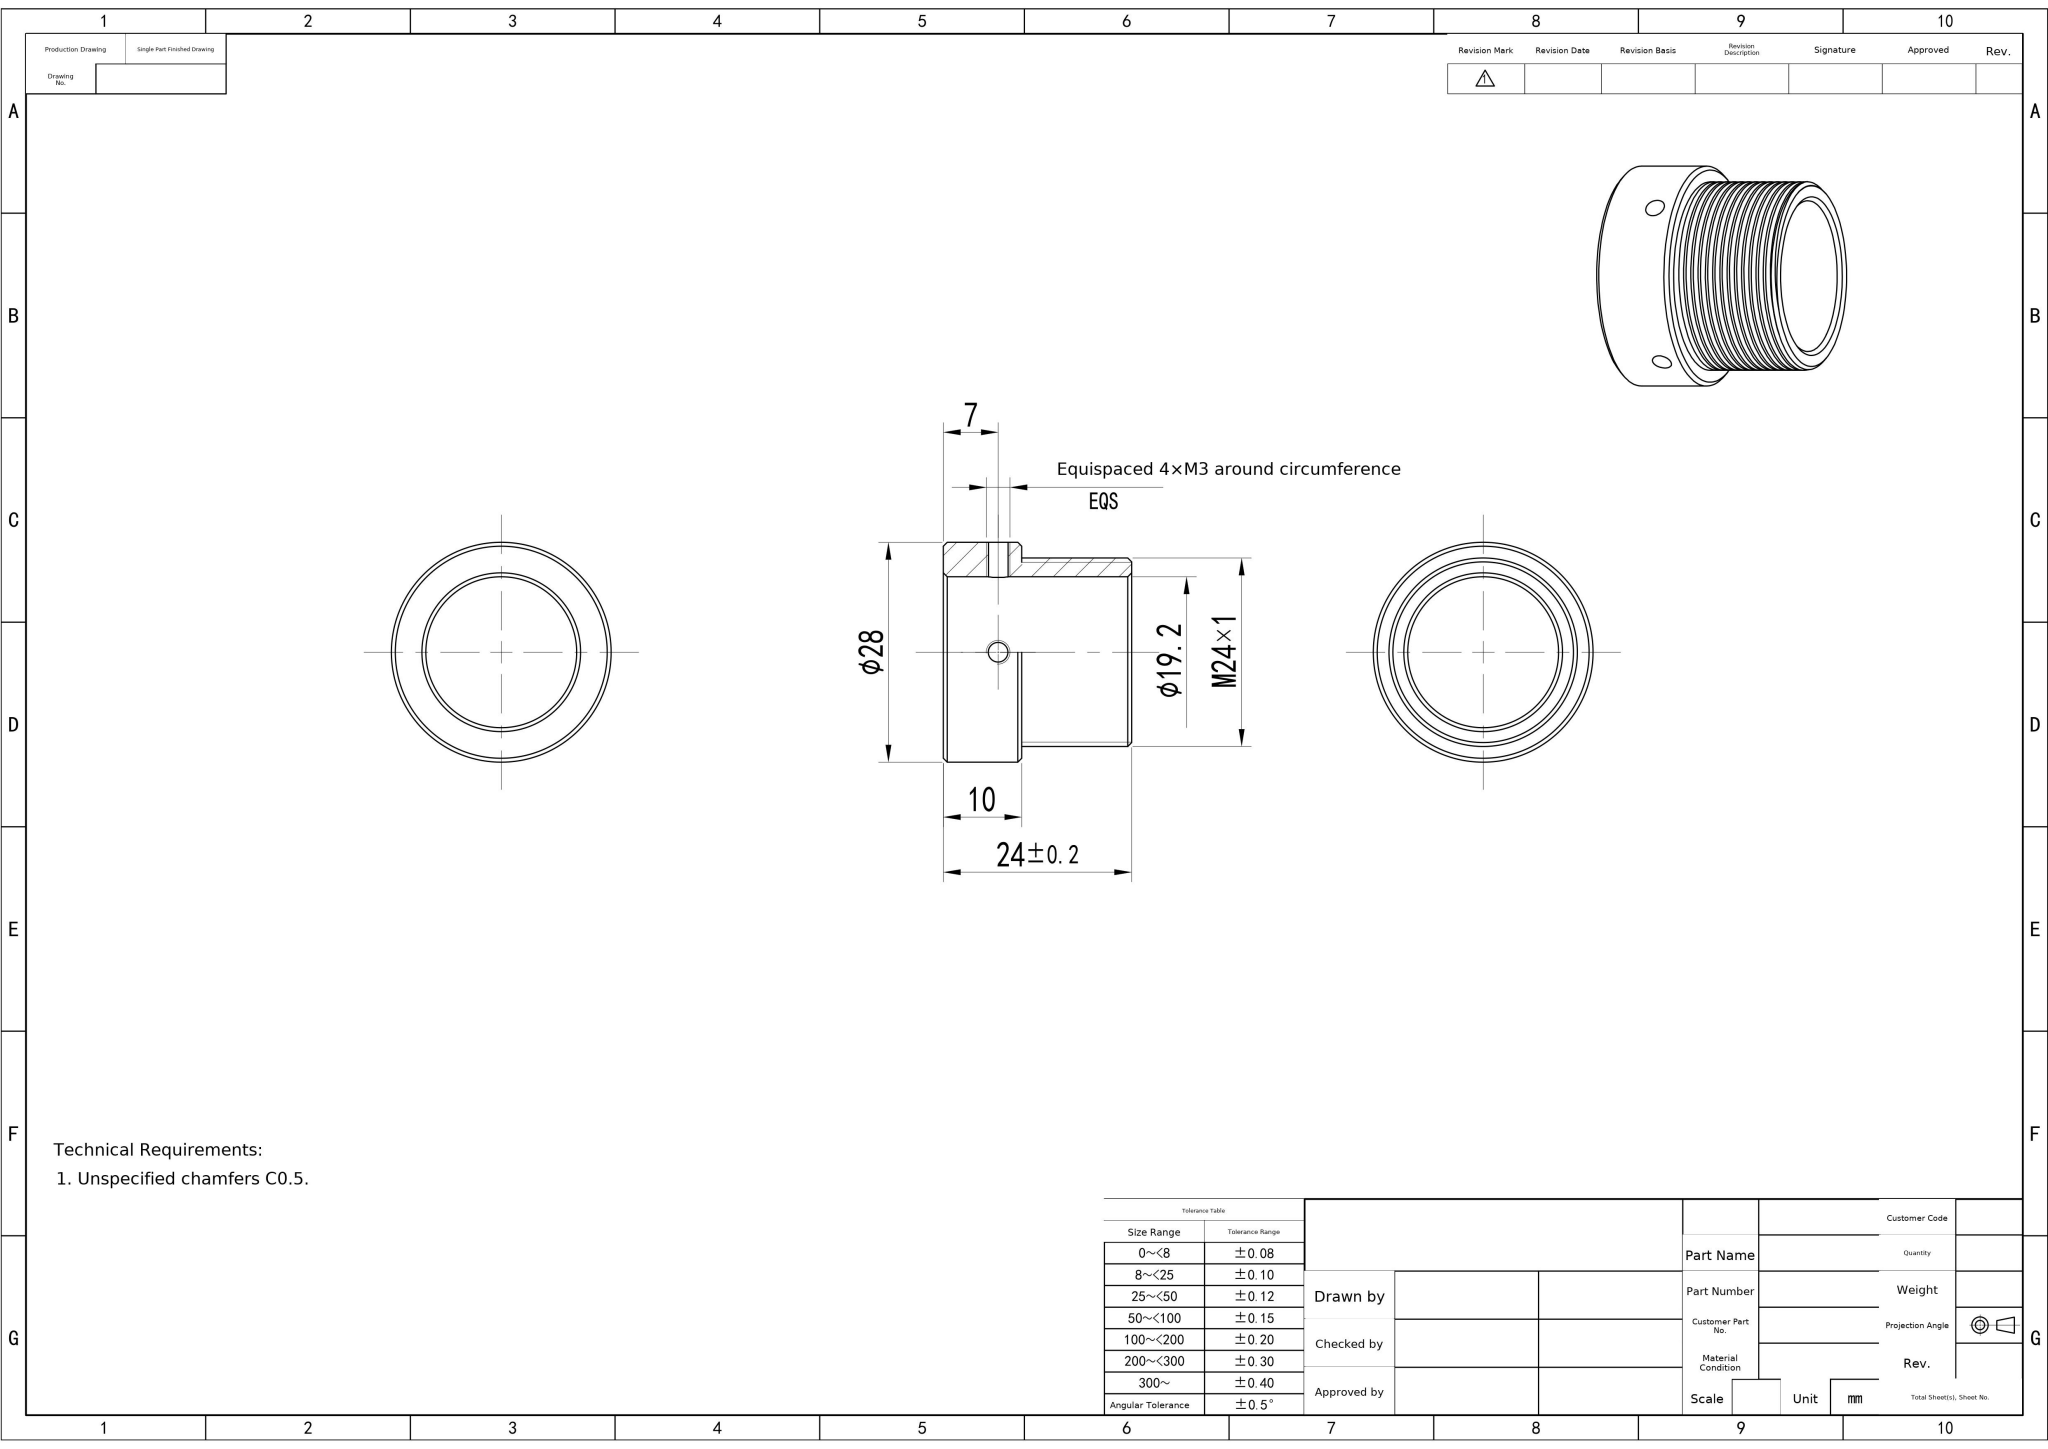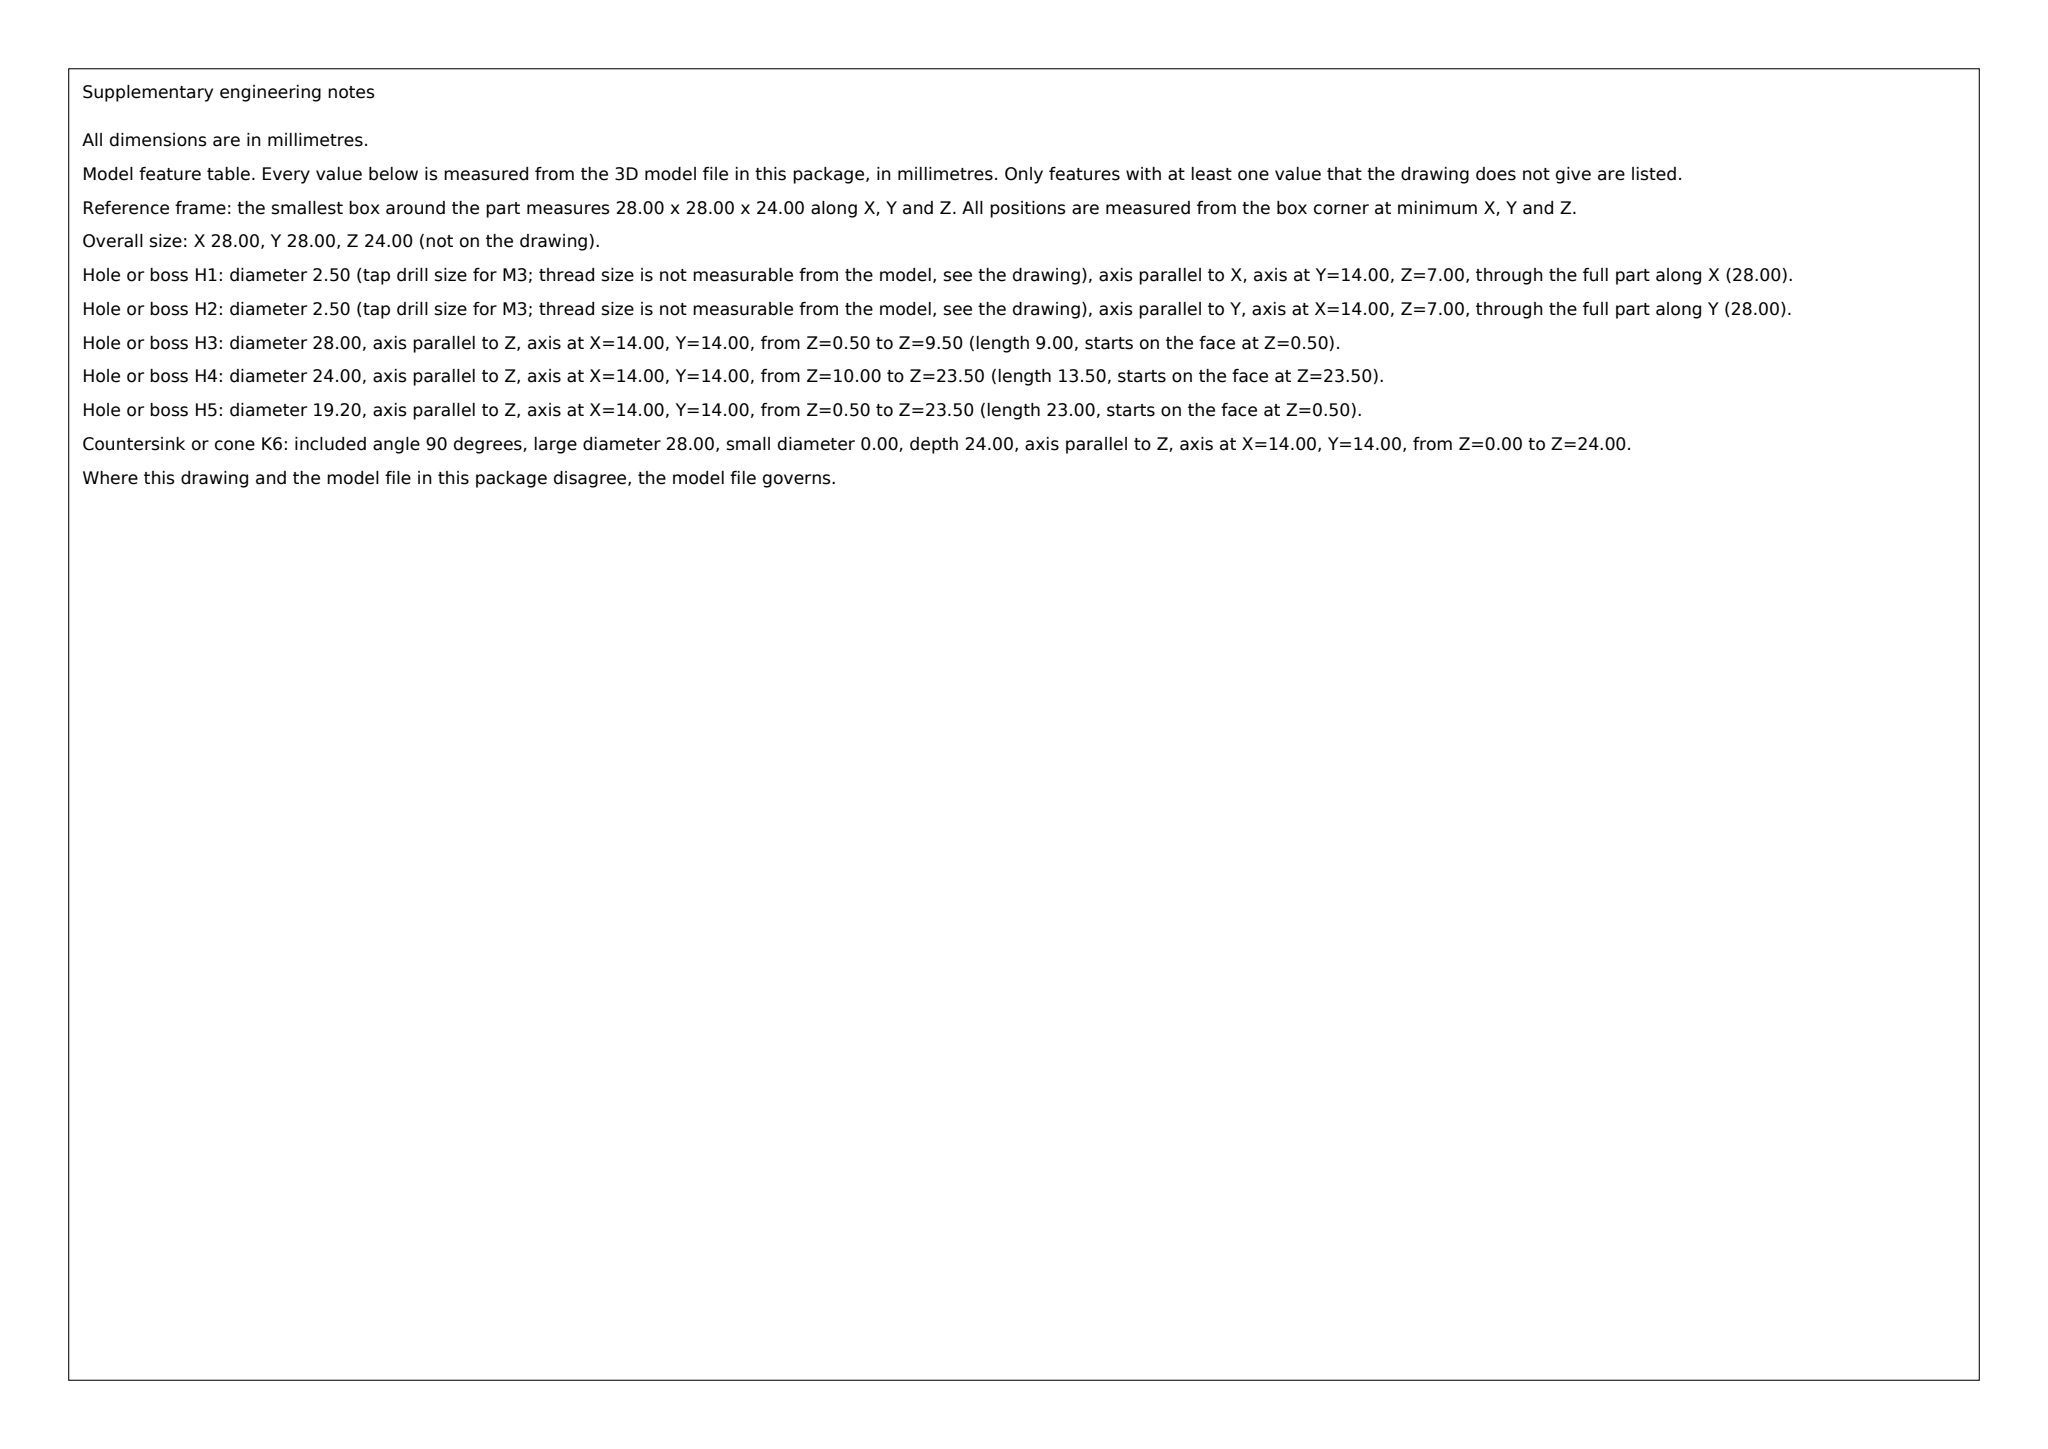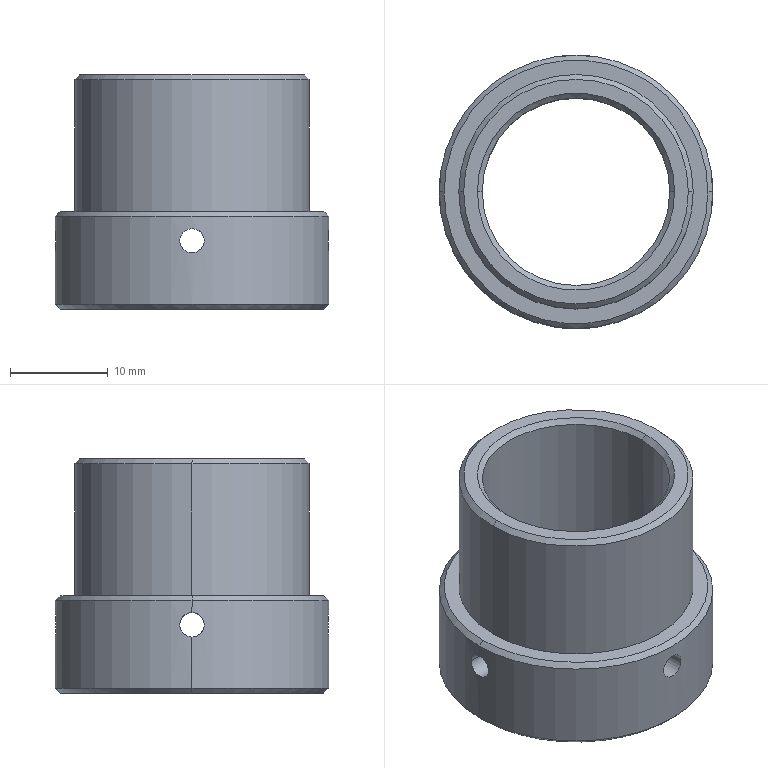Part | SolidWorks | mm | 1 solid | 27 faces | box 28 x 28 x 24 mm | volume 5409 mm3 | cylinder 14 | cone 10 | plane 3 | commonest cylinder face diameters 2.5 x8 19.2 x2 28 x2 24 x2